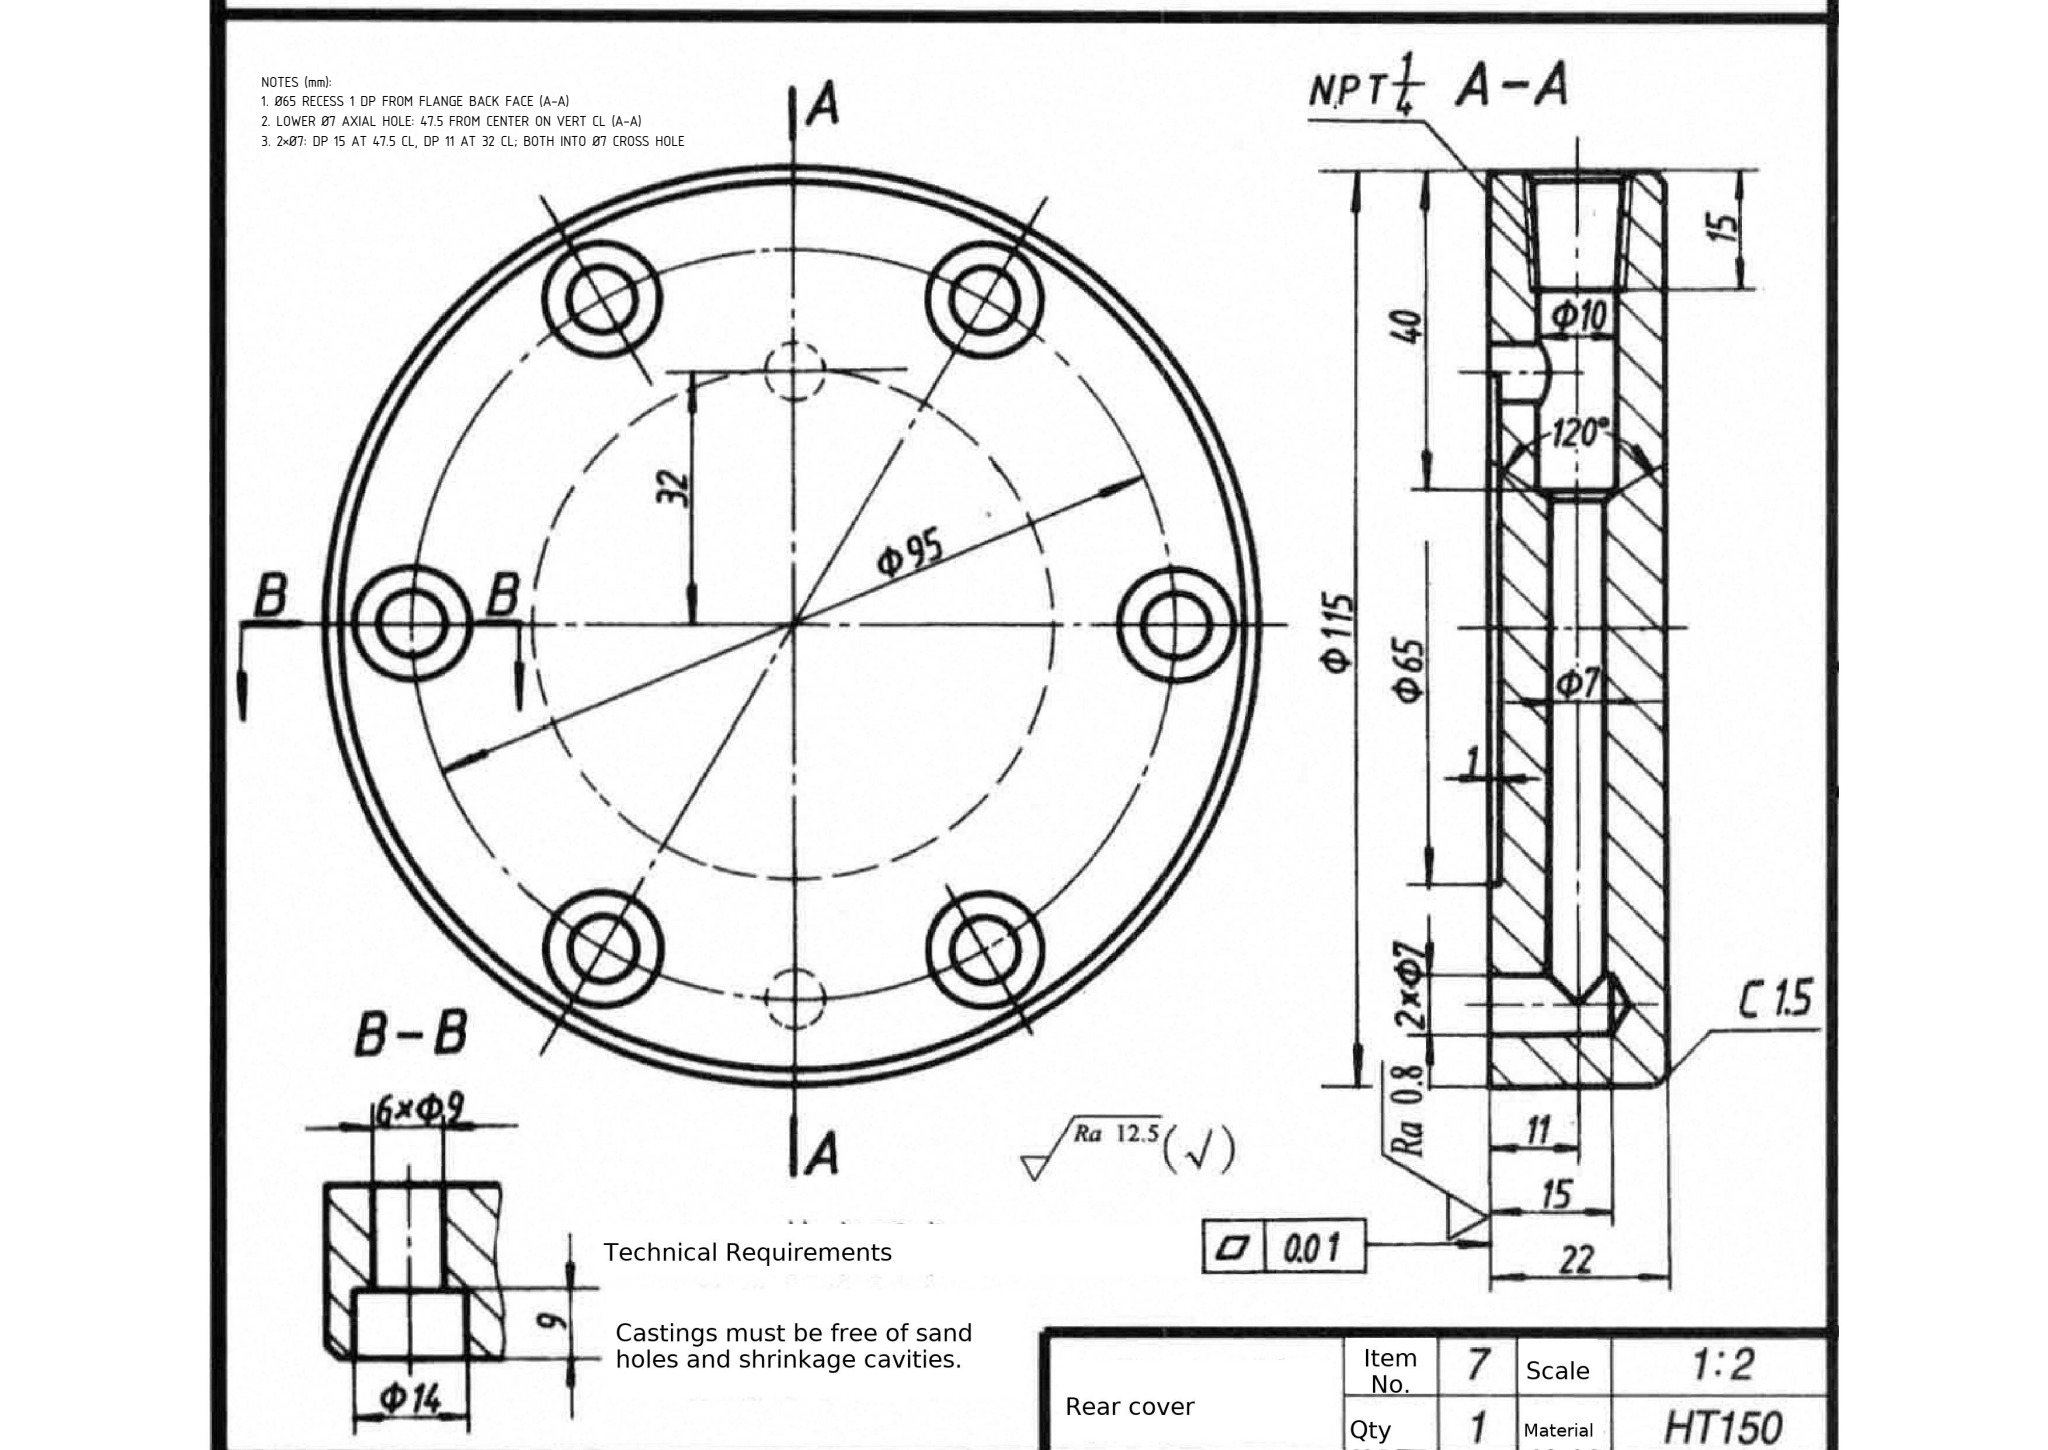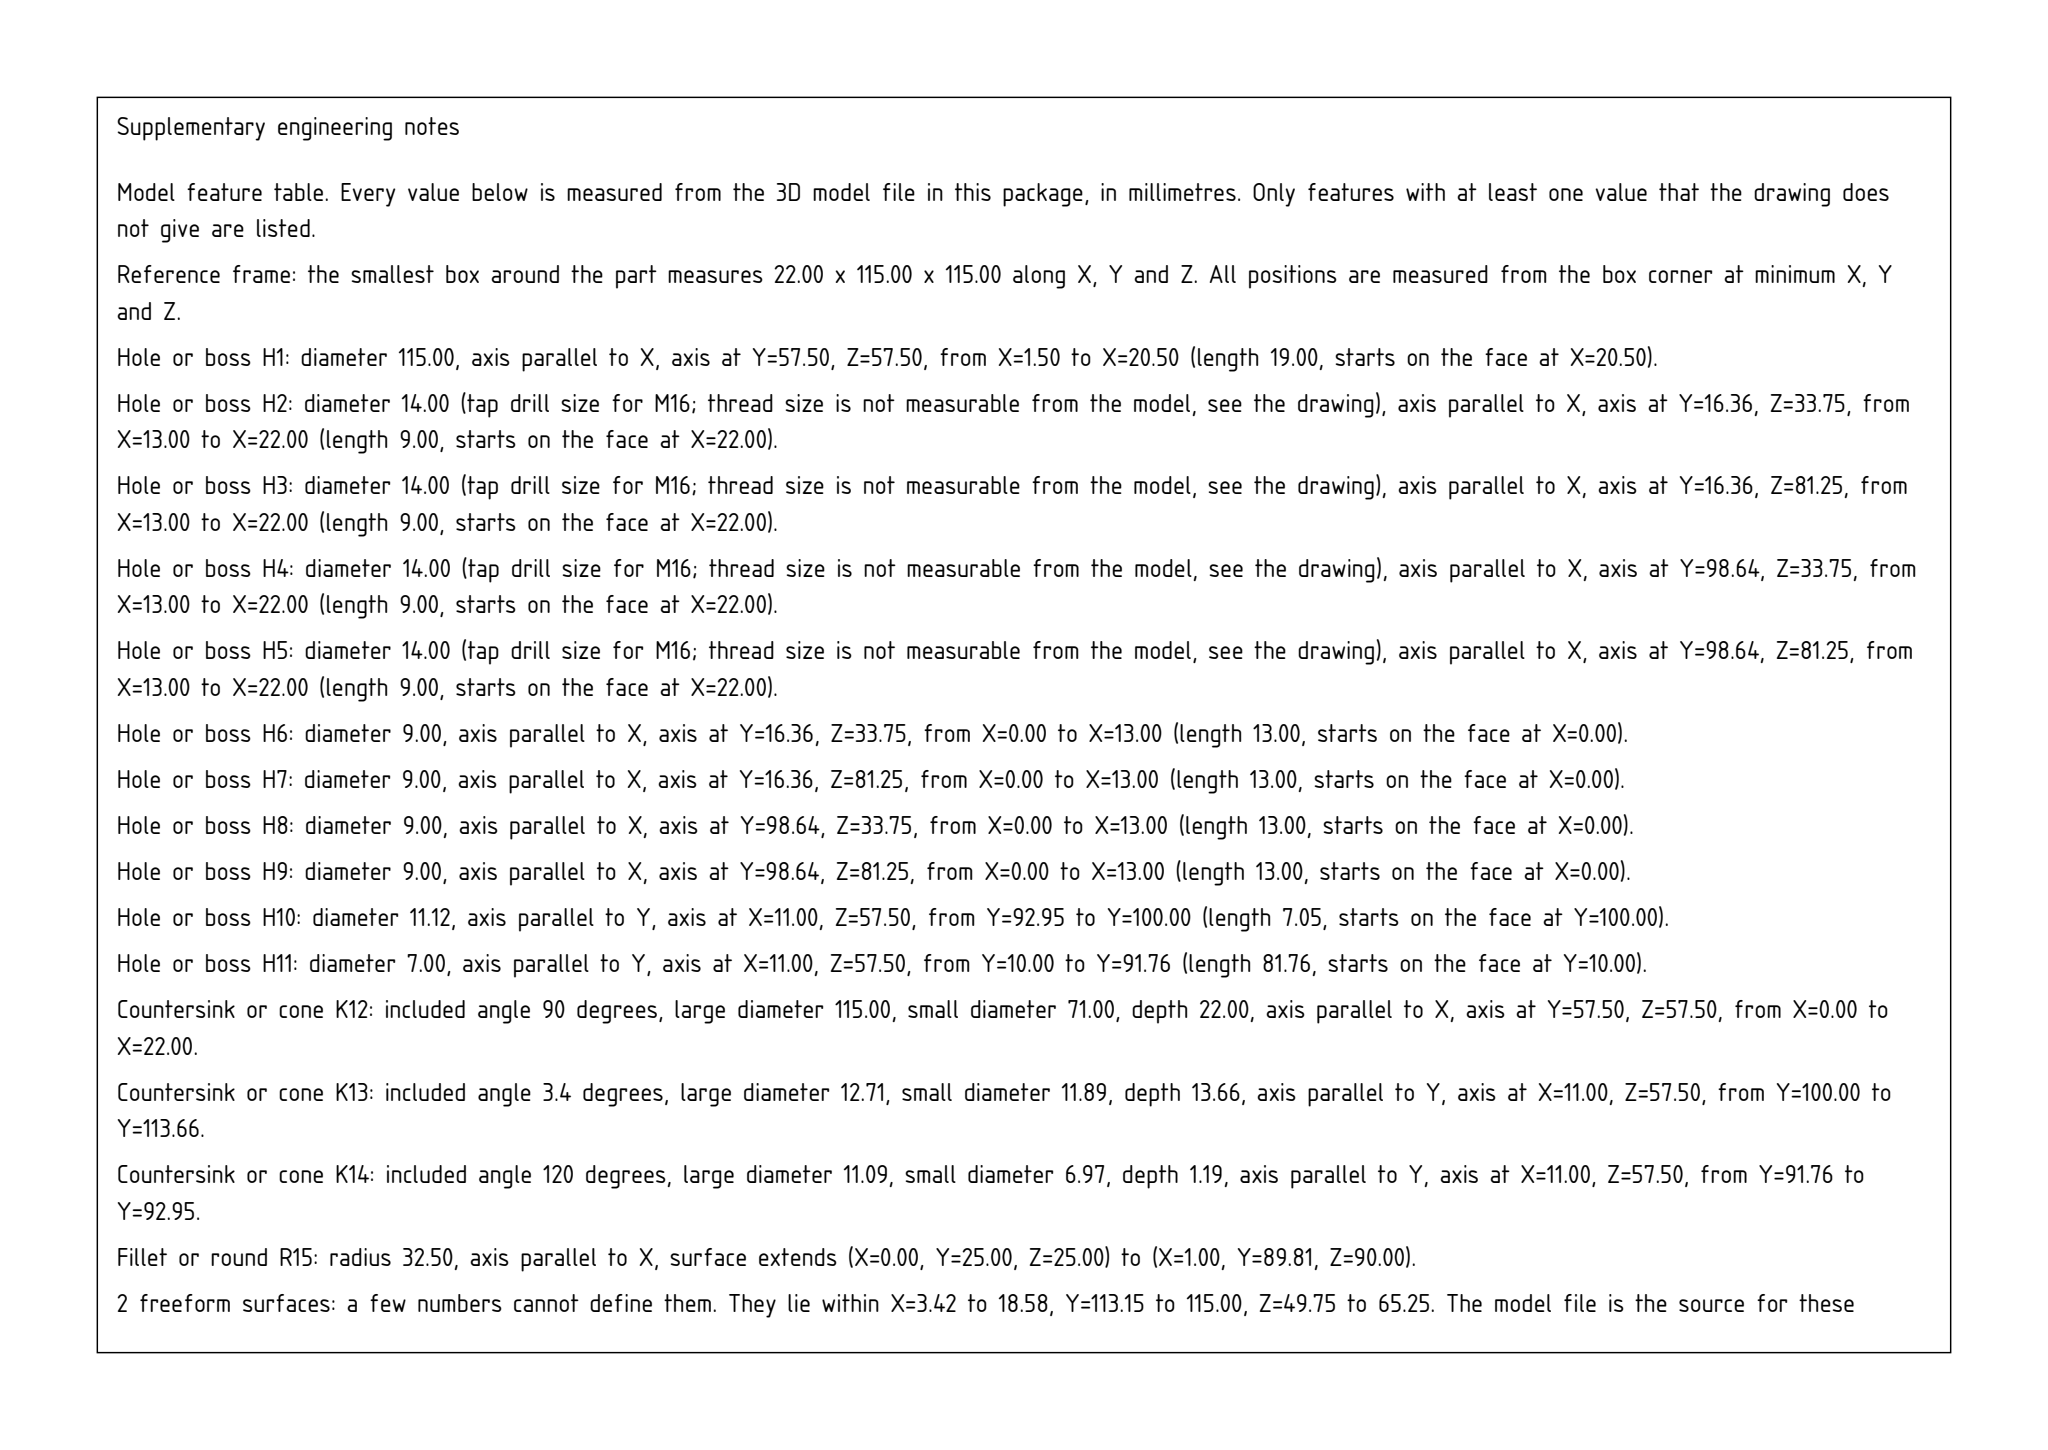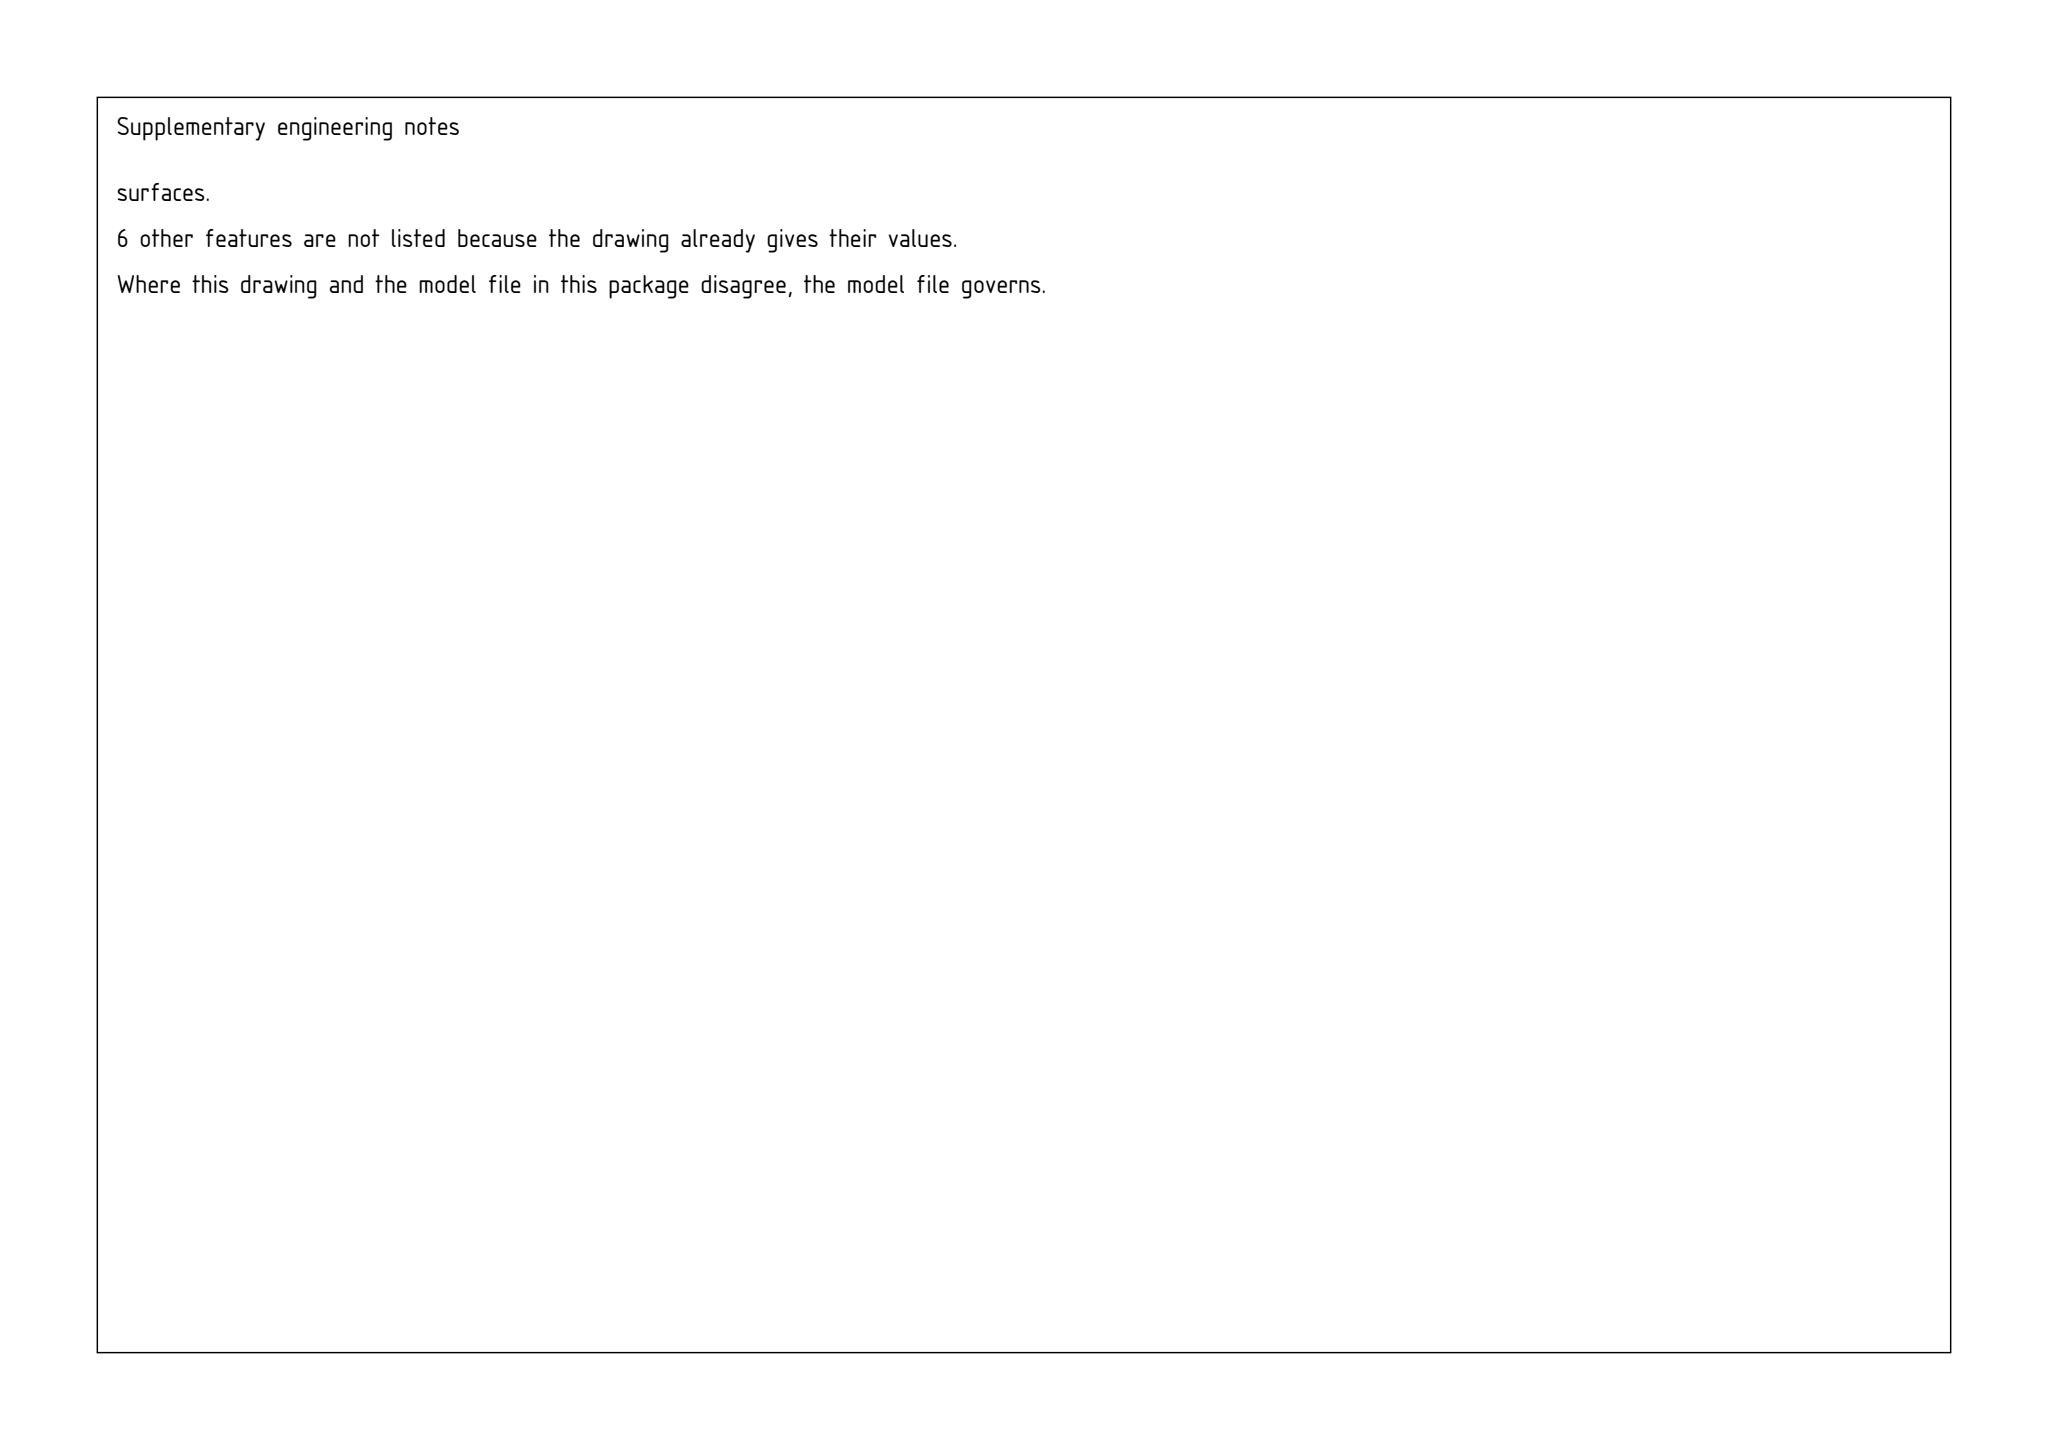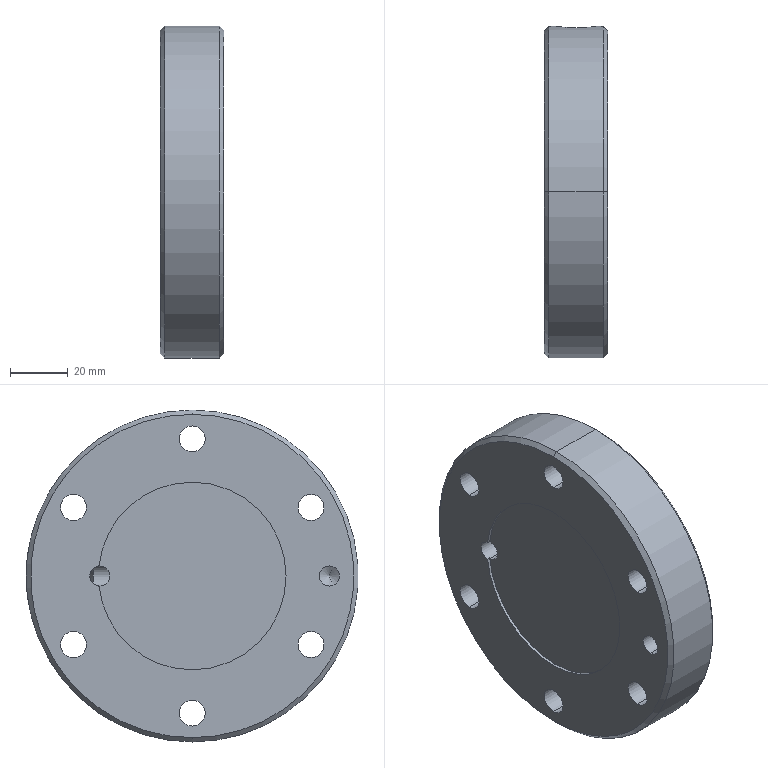Part | SolidWorks | mm | 1 solid | 63 faces | box 22 x 115 x 115 mm | volume 204610 mm3 | cylinder 40 | cone 11 | plane 10 | spline 2 | commonest cylinder face diameters 14 x12 9 x12 7 x9 65 x3 11.125 x2 115 x2
Drawing notes:
Ø65 RECESS 1 DP FROM FLANGE BACK FACE (A-A) | from the solid: Ø65 cylinder, axis x, length 1.0; x-planes at 0.0 and 1.0 (22 total thk)
LOWER Ø7 AXIAL HOLE: 47.5 FROM CENTER ON VERT CL (A-A) | from the solid: Ø7 x-axis holes at y=10 and y=89.5; part CL y=57.5 -> offsets 47.5 and 32
2×Ø7: DP 15 AT 47.5 CL, DP 11 AT 32 CL; BOTH INTO Ø7 CROSS HOLE | from the solid: Ø7 x-hole at y=10: faces 11+4=15 from x=0 face; Ø7 x-hole at y=89.5: face 11 (and 10 from Ø65x1 recess floor) ending at cross-hole axis x=11